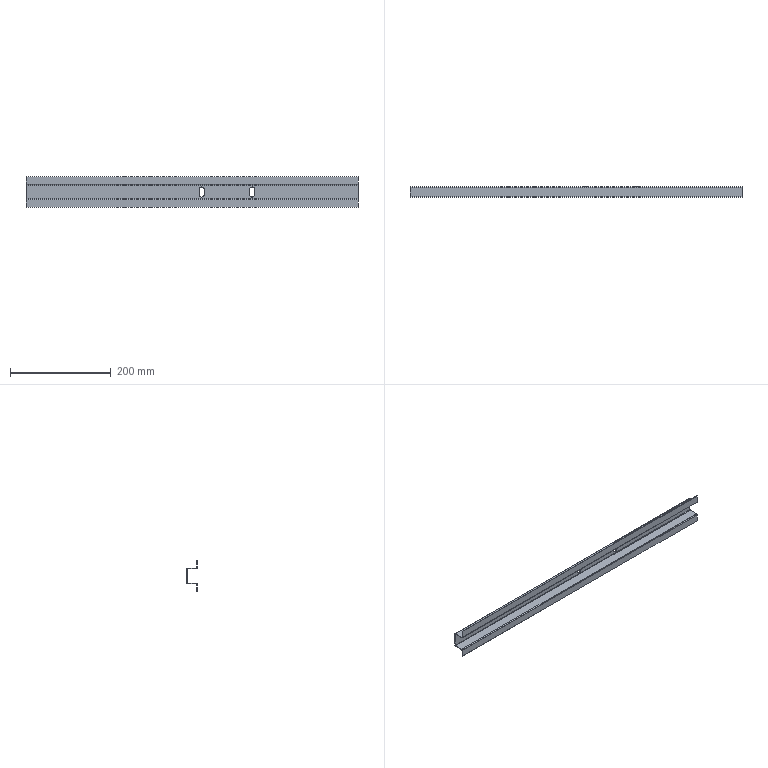Component | SolidWorks | CCQ-1.1-20Support2-1 | 1 solid | 48 faces | volume 64046 mm3 | plane 34 | cylinder 14 | commonest cylinder face diameters 10 x6 1.473 x4 3.473 x4 | material 304